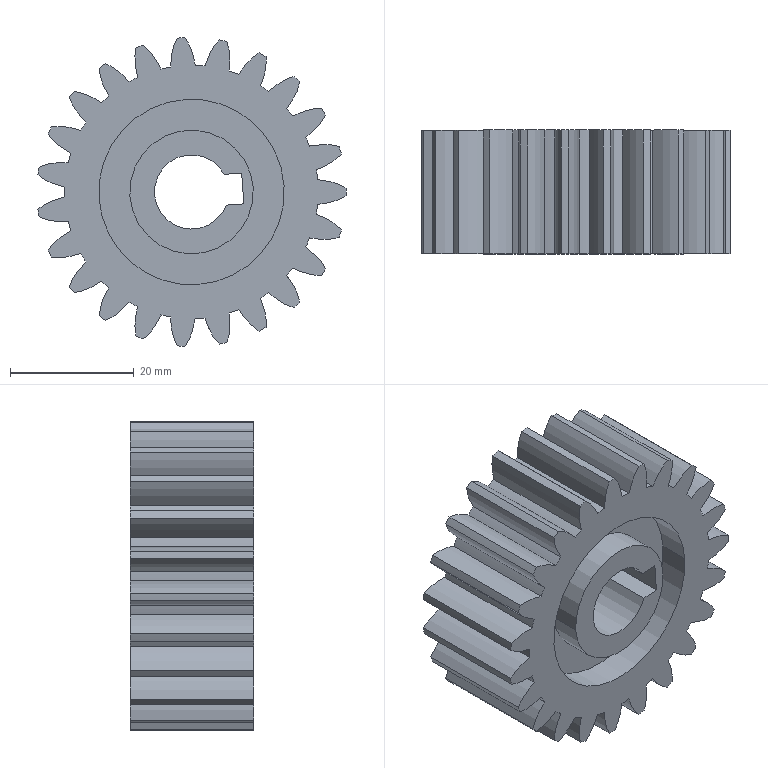Component | SolidWorks | 23-ToothGear-2 | 1 solid | 110 faces | volume 25094 mm3 | cylinder 55 | spline 46 | plane 9 | commonest cylinder face diameters 50 x23 41 x23 20 x4 30 x4 12 x1